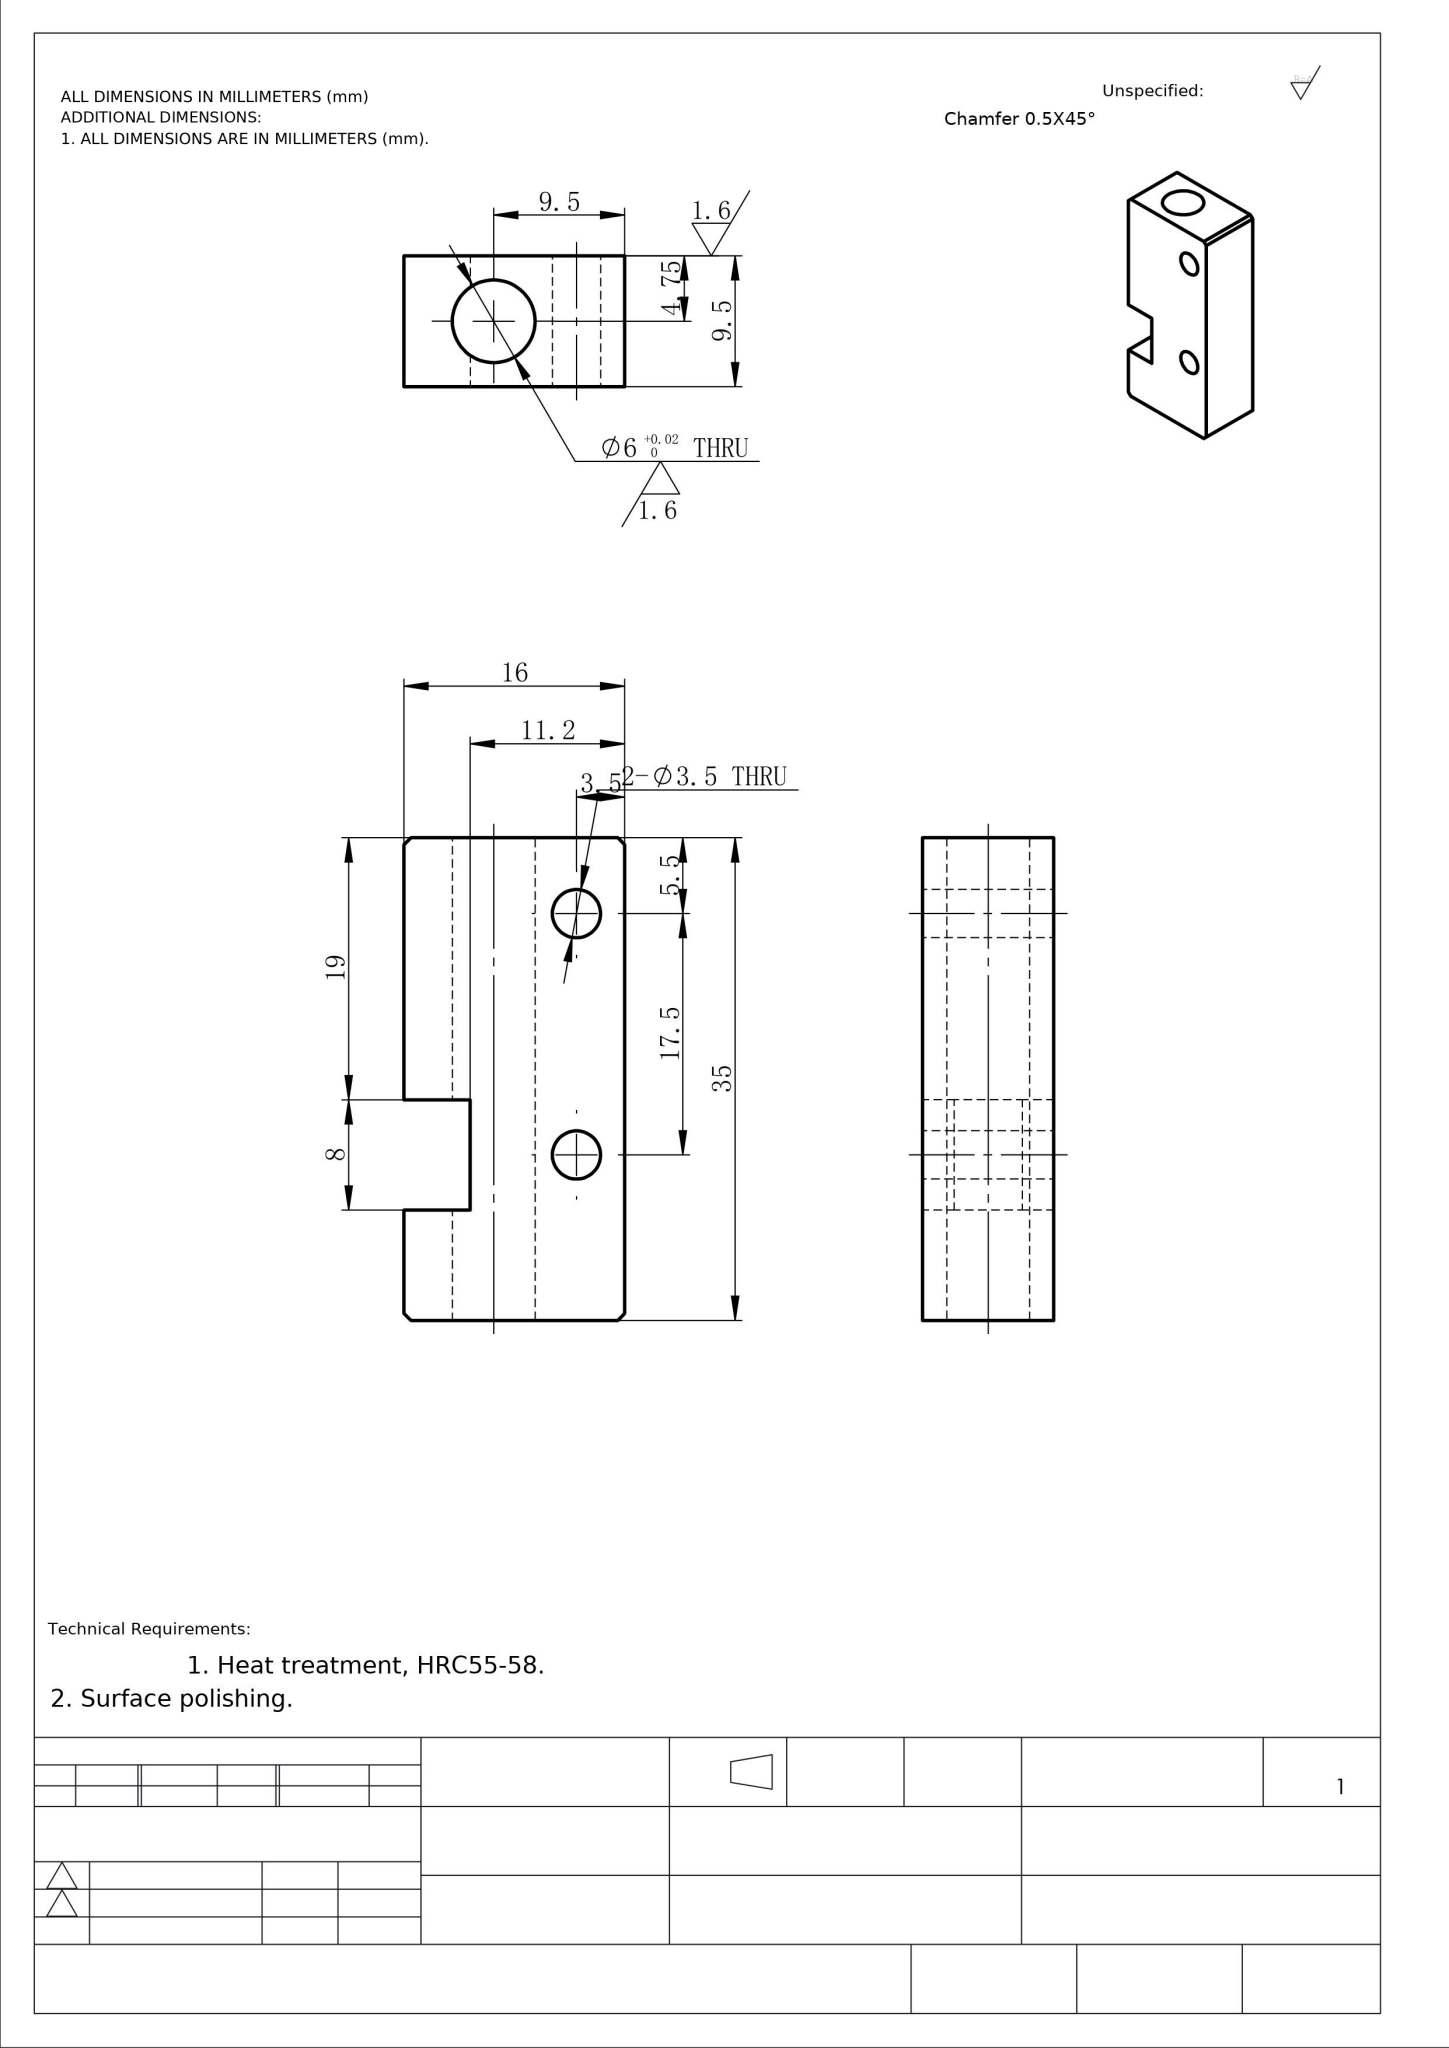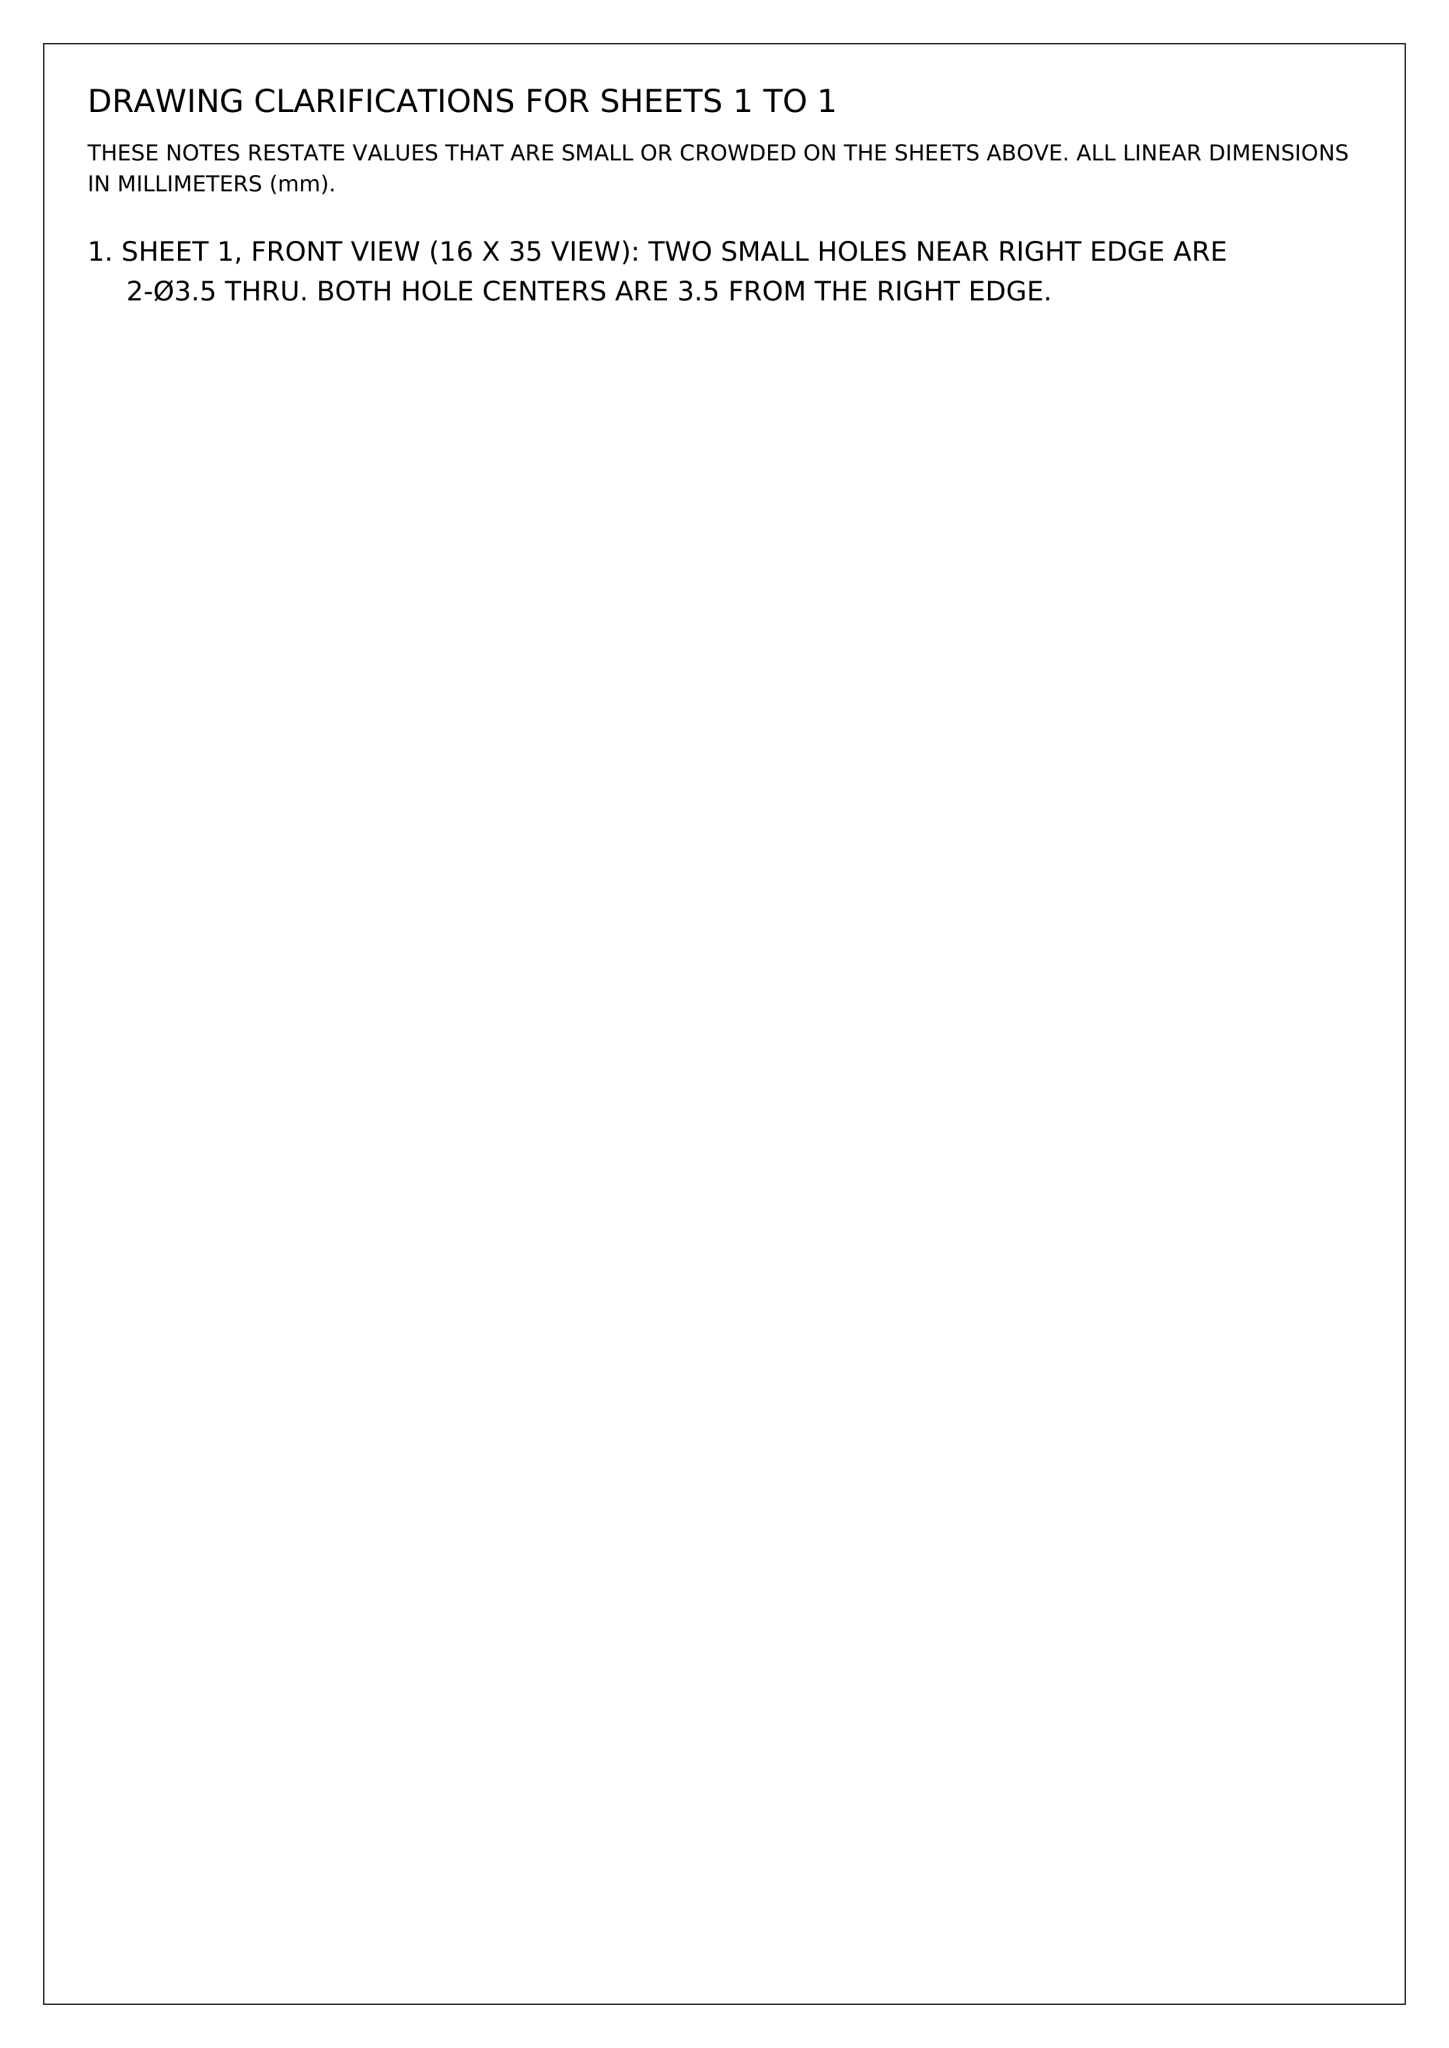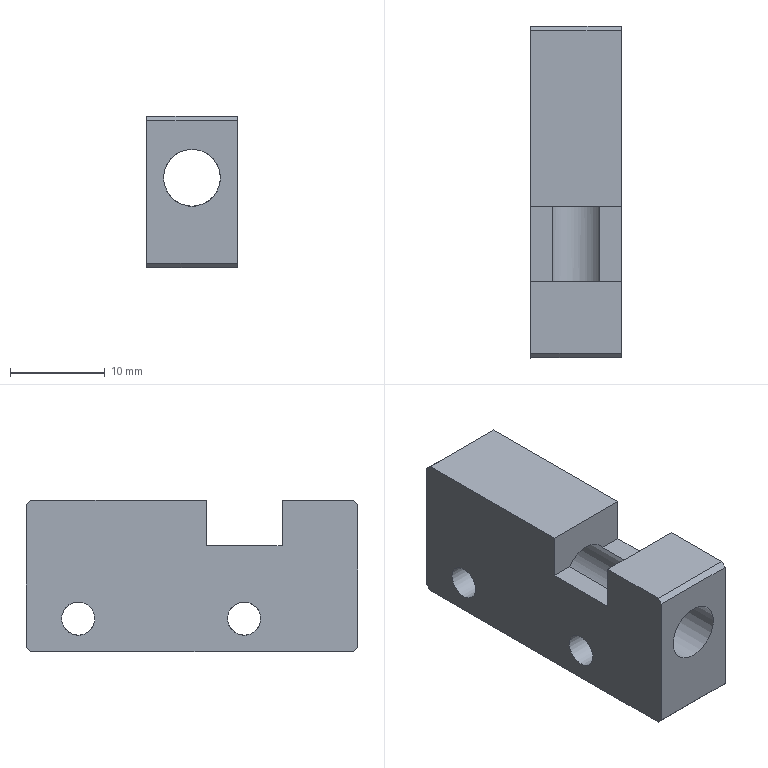Part | NX | mm | Stepped Twin-Block Bore Mount | 1 solid | 18 faces | box 9.5 x 35 x 16 mm | volume 3814 mm3 | plane 15 | cylinder 3 | commonest cylinder face diameters 3.5 x2 6 x1